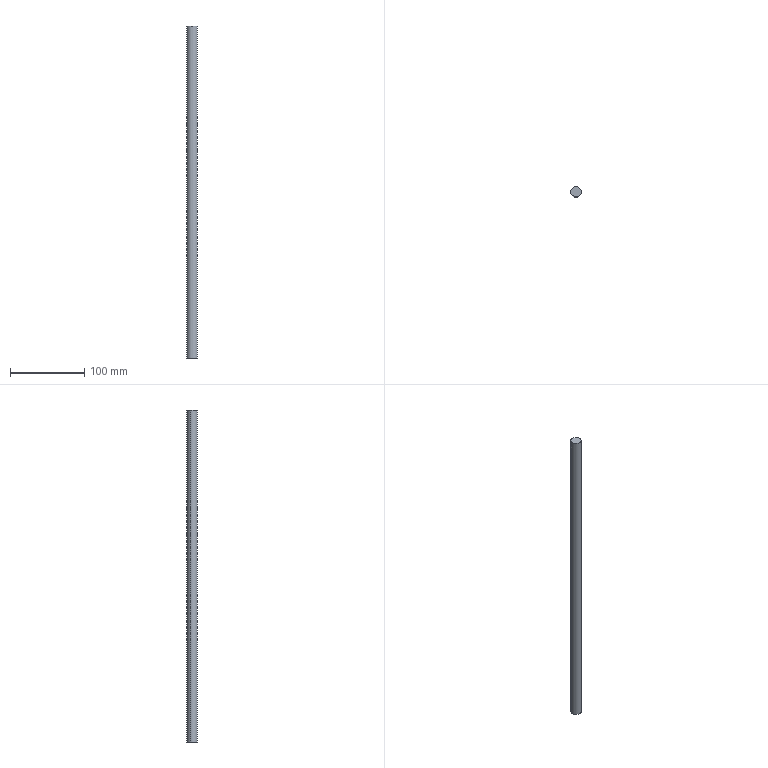Component | SolidWorks | Crossbar-1 | 1 solid | 4 faces | box 14 x 14 x 446 mm | volume 68656 mm3 | cylinder 2 | plane 2 | commonest cylinder face diameters 14 x2
build123d program:
from build123d import *

# Parameters (mm, degrees)
SKETCH1_W     = 8
SKETCH1_H     = 446
MOVE_FACE1_BY = 1


with BuildPart() as part:
    # Sketch1 → Revolve1 (revolve)
    with BuildSketch(Plane.XZ, mode=Mode.PRIVATE) as revolve1_sk:
        with Locations((4, 0)):
            Rectangle(SKETCH1_W, SKETCH1_H)
    revolve(revolve1_sk.sketch.rotate(Axis((0, 0, 223), (0, 0, -1)), 180), axis=Axis((0, 0, 223), (0, 0, -1)))

    # Move Face1: a curved face moved inward by 1.0
    add(Solid.thicken(part.faces().sort_by_distance((8, 0, 0))[0], -MOVE_FACE1_BY), mode=Mode.SUBTRACT)


solid = part.part

# Placed as in the assembly
solid = solid.moved(Location((-36, 125.451, -3.32), (0, 0, 0)))
STEP:
#1=COLOUR_RGB('',0.7922,0.8196,0.9333);
#2=FILL_AREA_STYLE_COLOUR('',#1);
#3=FILL_AREA_STYLE('',(#2));
#4=SURFACE_STYLE_FILL_AREA(#3);
#5=SURFACE_SIDE_STYLE('',(#4));
#6=SURFACE_STYLE_USAGE(.BOTH.,#5);
#7=PRESENTATION_STYLE_ASSIGNMENT((#6));
#8=CARTESIAN_POINT('',(-1.684,5.007,8.649));
#9=VERTEX_POINT('',#8);
#10=CARTESIAN_POINT('',(-1.15,4.871,8.649));
#11=VERTEX_POINT('',#10);
#12=CARTESIAN_POINT('',(-1.417,4.939,8.649));
#13=DIRECTION('',(-0.,-0.,-1.));
#14=DIRECTION('',(0.9692,-0.2464,0.));
#15=AXIS2_PLACEMENT_3D('',#12,#13,#14);
#16=CIRCLE('',#15,0.2756);
#17=EDGE_CURVE('',#9,#11,#16,.T.);
#18=ORIENTED_EDGE('',*,*,#17,.T.);
#19=CARTESIAN_POINT('',(-1.15,4.871,-8.91));
#20=VERTEX_POINT('',#19);
#21=CARTESIAN_POINT('',(-1.15,4.871,8.649));
#22=DIRECTION('',(-0.,-0.,-1.));
#23=VECTOR('',#22,39.37);
#24=LINE('',#21,#23);
#25=EDGE_CURVE('',#11,#20,#24,.T.);
#26=ORIENTED_EDGE('',*,*,#25,.T.);
#27=CARTESIAN_POINT('',(-1.684,5.007,-8.91));
#28=VERTEX_POINT('',#27);
#29=CARTESIAN_POINT('',(-1.417,4.939,-8.91));
#30=DIRECTION('',(-0.,-0.,-1.));
#31=DIRECTION('',(-0.9692,0.2464,0.));
#32=AXIS2_PLACEMENT_3D('',#29,#30,#31);
#33=CIRCLE('',#32,0.2756);
#34=EDGE_CURVE('',#28,#20,#33,.T.);
#35=ORIENTED_EDGE('',*,*,#34,.F.);
#36=CARTESIAN_POINT('',(-1.684,5.007,8.649));
#37=DIRECTION('',(-0.,-0.,-1.));
#38=VECTOR('',#37,39.37);
#39=LINE('',#36,#38);
#40=EDGE_CURVE('',#9,#28,#39,.T.);
#41=ORIENTED_EDGE('',*,*,#40,.F.);
#42=EDGE_LOOP('',(#18,#26,#35,#41));
#43=FACE_OUTER_BOUND('',#42,.T.);
#44=CARTESIAN_POINT('',(-1.417,4.939,8.649));
#45=DIRECTION('',(-0.,-0.,-1.));
#46=DIRECTION('',(-0.9692,0.2464,0.));
#47=AXIS2_PLACEMENT_3D('',#44,#45,#46);
#48=CYLINDRICAL_SURFACE('',#47,0.2756);
#49=ADVANCED_FACE('',(#43),#48,.T.);
#50=ORIENTED_EDGE('',*,*,#25,.F.);
#51=CARTESIAN_POINT('',(-1.417,4.939,8.649));
#52=DIRECTION('',(-0.,-0.,-1.));
#53=DIRECTION('',(0.9692,-0.2464,0.));
#54=AXIS2_PLACEMENT_3D('',#51,#52,#53);
#55=CIRCLE('',#54,0.2756);
#56=EDGE_CURVE('',#11,#9,#55,.T.);
#57=ORIENTED_EDGE('',*,*,#56,.T.);
#58=ORIENTED_EDGE('',*,*,#40,.T.);
#59=CARTESIAN_POINT('',(-1.417,4.939,-8.91));
#60=DIRECTION('',(-0.,-0.,-1.));
#61=DIRECTION('',(-0.9692,0.2464,0.));
#62=AXIS2_PLACEMENT_3D('',#59,#60,#61);
#63=CIRCLE('',#62,0.2756);
#64=EDGE_CURVE('',#20,#28,#63,.T.);
#65=ORIENTED_EDGE('',*,*,#64,.F.);
#66=EDGE_LOOP('',(#50,#57,#58,#65));
#67=FACE_OUTER_BOUND('',#66,.T.);
#68=CARTESIAN_POINT('',(-1.417,4.939,8.649));
#69=DIRECTION('',(-0.,-0.,-1.));
#70=DIRECTION('',(-0.9692,0.2464,0.));
#71=AXIS2_PLACEMENT_3D('',#68,#69,#70);
#72=CYLINDRICAL_SURFACE('',#71,0.2756);
#73=ADVANCED_FACE('',(#67),#72,.T.);
#74=ORIENTED_EDGE('',*,*,#17,.F.);
#75=ORIENTED_EDGE('',*,*,#56,.F.);
#76=EDGE_LOOP('',(#74,#75));
#77=FACE_OUTER_BOUND('',#76,.T.);
#78=CARTESIAN_POINT('',(-1.112,4.861,8.649));
#79=DIRECTION('',(0.,0.,1.));
#80=DIRECTION('',(0.9692,-0.2464,-0.));
#81=AXIS2_PLACEMENT_3D('',#78,#79,#80);
#82=PLANE('',#81);
#83=ADVANCED_FACE('',(#77),#82,.T.);
#84=ORIENTED_EDGE('',*,*,#34,.T.);
#85=ORIENTED_EDGE('',*,*,#64,.T.);
#86=EDGE_LOOP('',(#84,#85));
#87=FACE_OUTER_BOUND('',#86,.T.);
#88=CARTESIAN_POINT('',(-1.417,4.939,-8.91));
#89=DIRECTION('',(-0.,-0.,-1.));
#90=DIRECTION('',(-0.9692,0.2464,0.));
#91=AXIS2_PLACEMENT_3D('',#88,#89,#90);
#92=PLANE('',#91);
#93=ADVANCED_FACE('',(#87),#92,.T.);
#94=CLOSED_SHELL('',(#49,#73,#83,#93));
#95=MANIFOLD_SOLID_BREP('',#94);
#96=STYLED_ITEM('',(#7),#95);
#97=PRESENTATION_LAYER_ASSIGNMENT('','',(#96));
#98=CARTESIAN_POINT('',(0.,0.,0.));
#99=DIRECTION('',(0.,0.,1.));
#100=DIRECTION('',(1.,0.,0.));
#101=AXIS2_PLACEMENT_3D('',#98,#99,#100);
#102=(LENGTH_UNIT()NAMED_UNIT(*)SI_UNIT($,.METRE.));
#103=LENGTH_MEASURE_WITH_UNIT(LENGTH_MEASURE(0.0254),#102);
#104=DIMENSIONAL_EXPONENTS(1.,0.,0.,0.,0.,0.,0.);
#105=(CONVERSION_BASED_UNIT('',#103)LENGTH_UNIT()NAMED_UNIT(#104));
#106=UNCERTAINTY_MEASURE_WITH_UNIT(LENGTH_MEASURE(0.00001),#105,'','');
#107=(NAMED_UNIT(*)PLANE_ANGLE_UNIT()SI_UNIT($,.RADIAN.));
#108=(NAMED_UNIT(*)SI_UNIT($,.STERADIAN.)SOLID_ANGLE_UNIT());
#109=(GEOMETRIC_REPRESENTATION_CONTEXT(3)GLOBAL_UNCERTAINTY_ASSIGNED_CONTEXT((#106))GLOBAL_UNIT_ASSIGNED_CONTEXT((#105,#107,#108))REPRESENTATION_CONTEXT('',''));
#110=ADVANCED_BREP_SHAPE_REPRESENTATION('',(#95,#101),#109);
#111=(LENGTH_UNIT()NAMED_UNIT(*)SI_UNIT($,.METRE.));
#112=LENGTH_MEASURE_WITH_UNIT(LENGTH_MEASURE(0.0254),#111);
#113=DIMENSIONAL_EXPONENTS(1.,0.,0.,0.,0.,0.,0.);
#114=(CONVERSION_BASED_UNIT('',#112)LENGTH_UNIT()NAMED_UNIT(#113));
#115=UNCERTAINTY_MEASURE_WITH_UNIT(LENGTH_MEASURE(0.00001),#114,'','');
#116=(NAMED_UNIT(*)PLANE_ANGLE_UNIT()SI_UNIT($,.RADIAN.));
#117=(NAMED_UNIT(*)SI_UNIT($,.STERADIAN.)SOLID_ANGLE_UNIT());
#118=(GEOMETRIC_REPRESENTATION_CONTEXT(3)GLOBAL_UNCERTAINTY_ASSIGNED_CONTEXT((#115))GLOBAL_UNIT_ASSIGNED_CONTEXT((#114,#116,#117))REPRESENTATION_CONTEXT('',''));
#119=MECHANICAL_DESIGN_GEOMETRIC_PRESENTATION_REPRESENTATION('',(#96),#118);